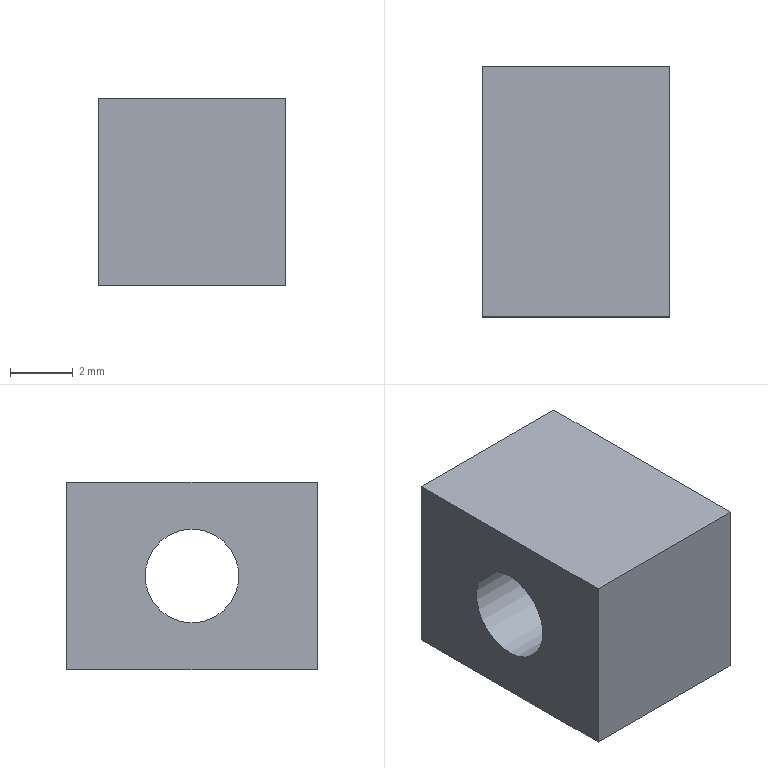Component | NX | LINK_6_BLOCK | 1 solid | 7 faces | volume 246 mm3 | plane 6 | cylinder 1 | commonest cylinder face diameters 3 x1